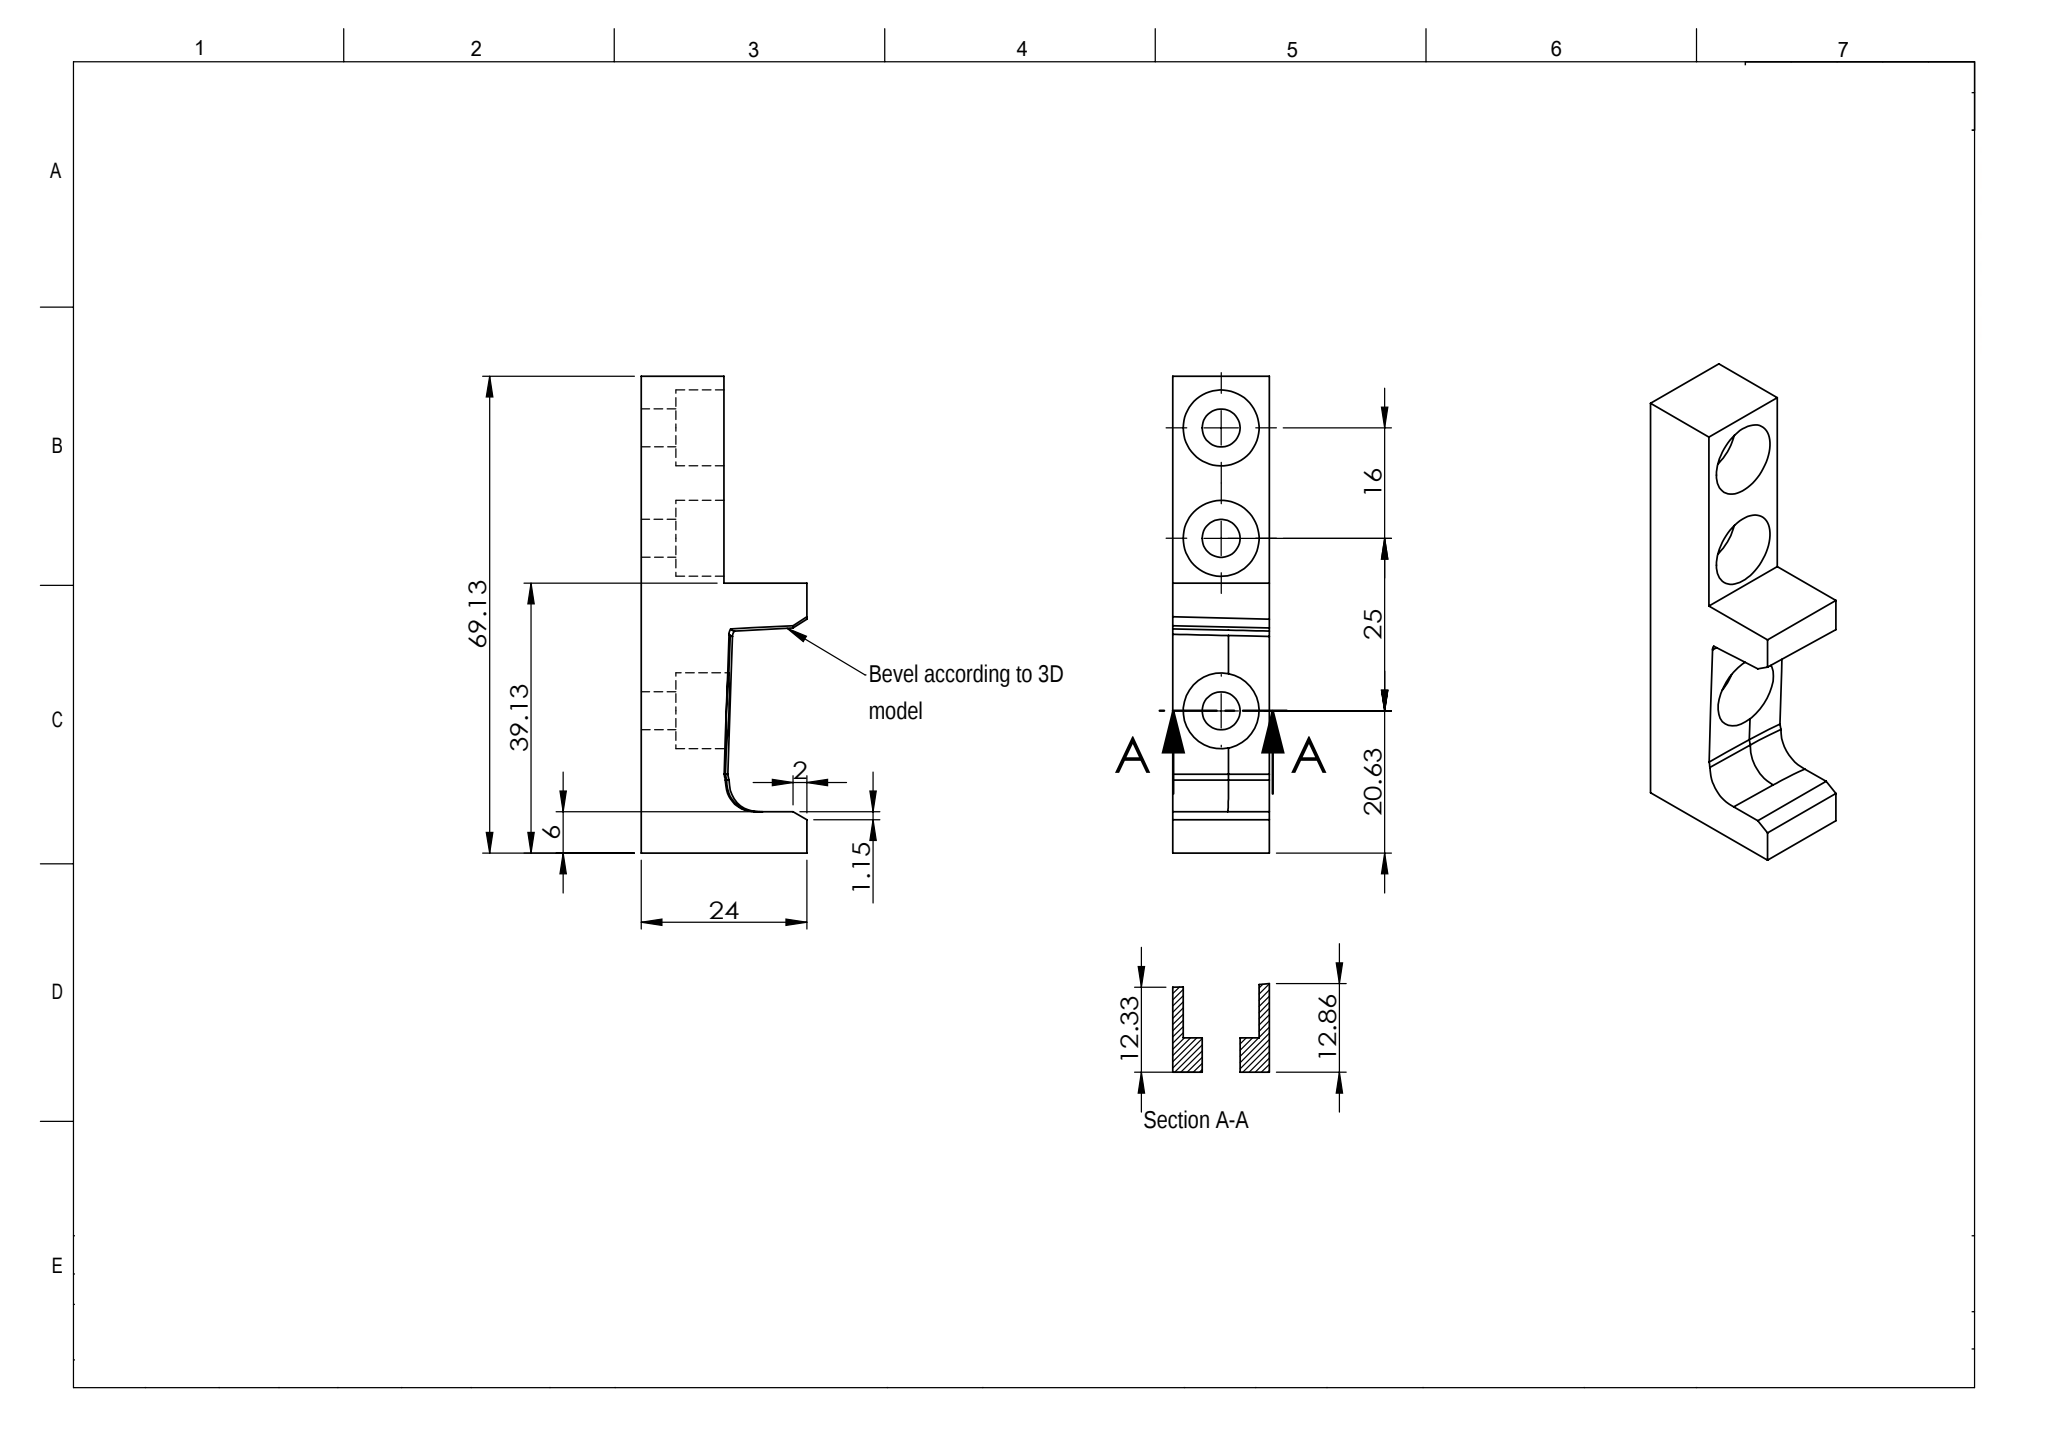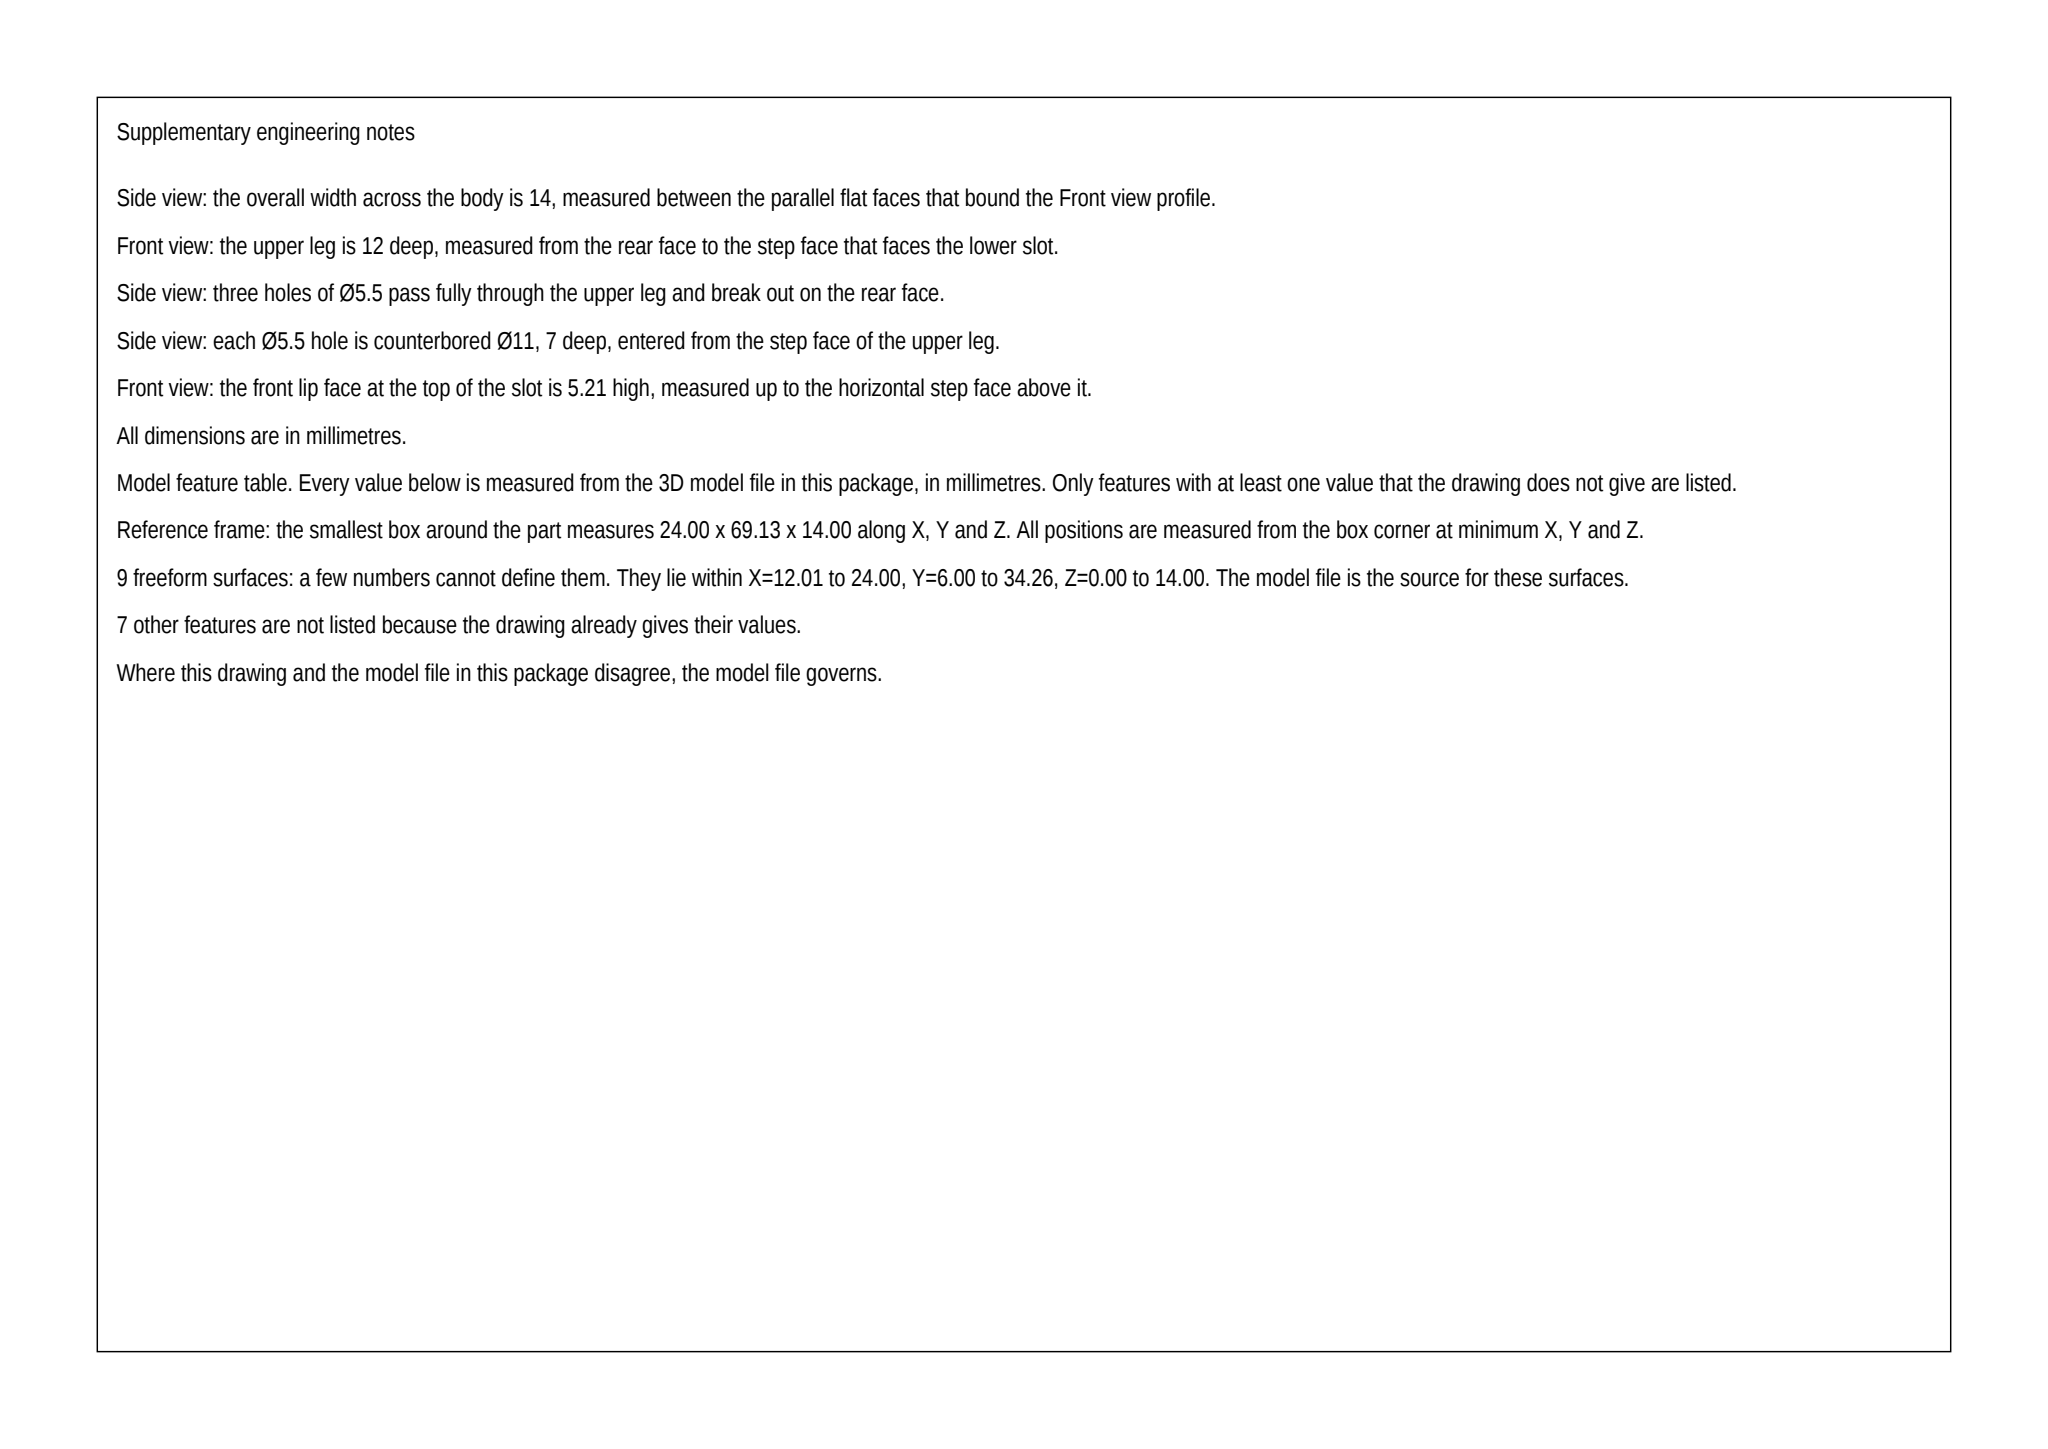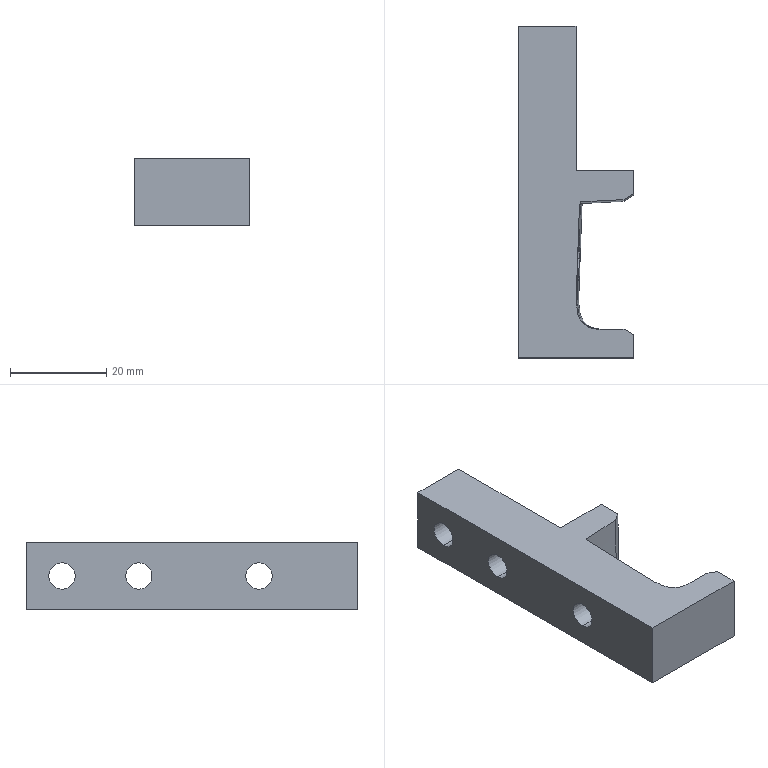Part | SolidWorks | mm | 1 solid | 35 faces | box 24 x 69.13 x 14 mm | volume 11531 mm3 | plane 14 | cylinder 12 | spline 9 | commonest cylinder face diameters 11 x6 5.5 x6